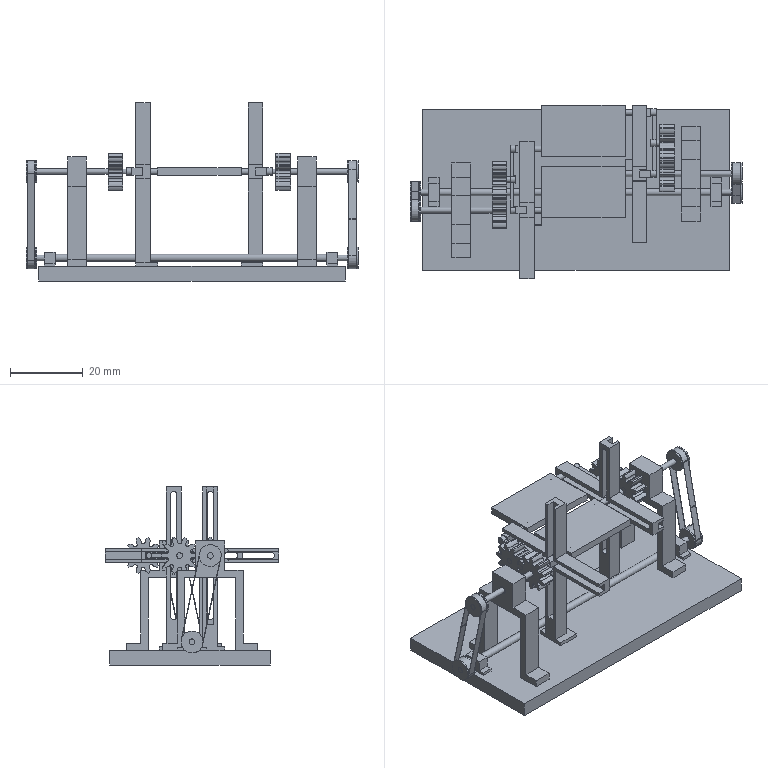Assembly | NX | mm | 28 component files | 30 solids | 595 faces | box 91 x 47.6 x 48.8 mm | volume 21339 mm3 | plane 280 | spline 212 | cylinder 83 | torus 20 | commonest cylinder face diameters 1.6 x42 6 x12 2 x11 0.02 x10 5.8 x8
Bill of materials:
unnamed part 1 | 2 |  | Straight-toothed spur-gear-like disc with about 10 rounded teeth and a plain central round bore; prismatic face width.
unnamed part 2 | 2 |  | Flat rectangular plate with one small round hole entering one of its short edge faces.
unnamed part 3 | 2 |  | Block shaped like an upside-down T: a raised rectangular boss with a horizontal through bore, sitting on a wider base with a flange on each side.
unnamed part 4 | 2 |  | Solid stepped cylindrical shaft with one short larger-diameter collar section placed off-center along its length.
unnamed part 5 | 2 |  | Cross-shaped frame made of two crossing bars, each with a long slot, joined at the center, with a small flat base plate at the bottom of the vertical bar.
unnamed part 6 | 2 |  | Straight-toothed spur-gear-like disc with about 10 rounded teeth and a plain central round bore.
unnamed part 7 | 4 |  | Cylindrical roller or pulley body with a slightly raised rim at each end and a central bore with one rectangular keyway.
unnamed part 8 | 2 |  | Bracket of constant thickness shaped like an arch or upside-down U, with outward-turned feet at the bottom and a rectangular tab on top holding a small round through hole.
unnamed part 9 | 2 |  | Thin-walled closed obround (stadium-shaped) loop band with an open center, like a flat belt or ring strap.
unnamed part 10 | 1 |  | Long slender solid rod with a short reduced-diameter step at each end.
unnamed part 11 | 2 |  | Straight bar with a hollow ring eye at each end and a central cylindrical boss carrying a perpendicular solid cylindrical pin.
unnamed part 12 | 1 |  | Plain thin flat rectangular plate with no visible holes or features.
unnamed part 13 | 4 |  | Straight solid cylindrical rod with a rectangular block of square cross-section fixed on it, coaxial with the rod and closer to one end. A long length of rod sticks out from one side of the block and a short stub from the other. Both rod ends are flat.
Mates:
1. touch align | gear_1 1 | gear_2 1
2. fix | base_plate 1 component
3. touch align | belt_shaft_2 1 face | belt 2 face
4. touch align | round_transfer 1 face | belt 2 face
5. touch align | belt_shaft_2 1 face | top 2 face
6. touch align | long_shaft 1 face | lower_fixed_shaft 2 face
7. touch align | round_transfer 2 face | long_shaft 1 face
8. touch align | belt 2 face | long_shaft 1 face
9. touch align | gear_set_2 2 face | belt_shaft_2 1 face
10. touch align | connecting_shaft_part 1 face | gear_set_2 2 face
11. touch align | mid_rect_2_circ 1 face | cross 2 face
12. touch align | top 2 face | base_plate 1 face
13. touch align | cross 2 face | base_plate 1 face
14. touch align | connecting_rect 1 face | mid_rect_2_circ 2 face
15. touch align | connecting_rect 2 face | mid_rect_2_circ 1 face
16. parallel | connecting_rect 2 face | base_plate 1 face
17. parallel | mid_rect_2_circ 2 face | base_plate 1 face
18. parallel | mid_rect_2_circ 1 face | base_plate 1 face
19. parallel | connecting_shaft_part 1 face | base_plate 1 face
20. touch align | connecting_shaft_part 1 face | connecting_shaft_part 2 face
21. concentric | mid_rect_2_circ 2 edge | connecting_shaft_part 1 edge
22. parallel | mid_rect_2_circ 1 face | base_plate 1 face
23. parallel | mid_rect_2_circ 2 face | base_plate 1 face
24. parallel | mid_rect_2_circ 2 face | base_plate 1 face
25. parallel | mid_rect_2_circ 1 face | base_plate 1 face
26. touch align | mid_rect_2_circ 3 face | connecting_rect 1 face
27. parallel | connecting_shaft_part 2 face | base_plate 1 face
28. touch align | connecting_shaft_part 2 face | mid_rect_2_circ 3 face
29. touch align | mid_rect_2_circ 4 face | connecting_shaft_part 2 face
30. touch align | mid_rect_2_circ 1 face | connecting_shaft_part 1 face
31. touch align | gear_set_2 1 face | connecting_shaft_part 2 face
32. parallel | mid_rect_2_circ 4 face | base_plate 1 face
33. distance | gear_set_2 2 face | belt_shaft_2 1 face
34. distance | gear_set_2 1 face | connecting_shaft_part 2 face
35. distance | connecting_shaft_part 2 face | base_plate 1 face
36. distance | gear_set_2 2 face | base_plate 1 face
37. distance | gear_set_2 2 face | base_plate 1 face
38. distance | gear_set_2 1 face | base_plate 1 face
39. touch align | cross 2 face | mid_rect_2_circ 1 face
40. touch align | cross 1 face | mid_rect_2_circ 4 face
41. touch align | belt_shaft_2 2 face | gear_set_2 1 face
42. touch align | top 1 face | belt_shaft_2 2 face
43. touch align | round_transfer 3 face | belt_shaft_2 2 face
44. touch align | round_transfer 4 face | long_shaft 1 face
45. concentric | belt 1 edge | round_transfer 3 edge
46. concentric | belt 1 edge | round_transfer 4 edge
47. touch align | lower_fixed_shaft 1 face | long_shaft 1 face
48. parallel | top 1 face | base_plate 1 face